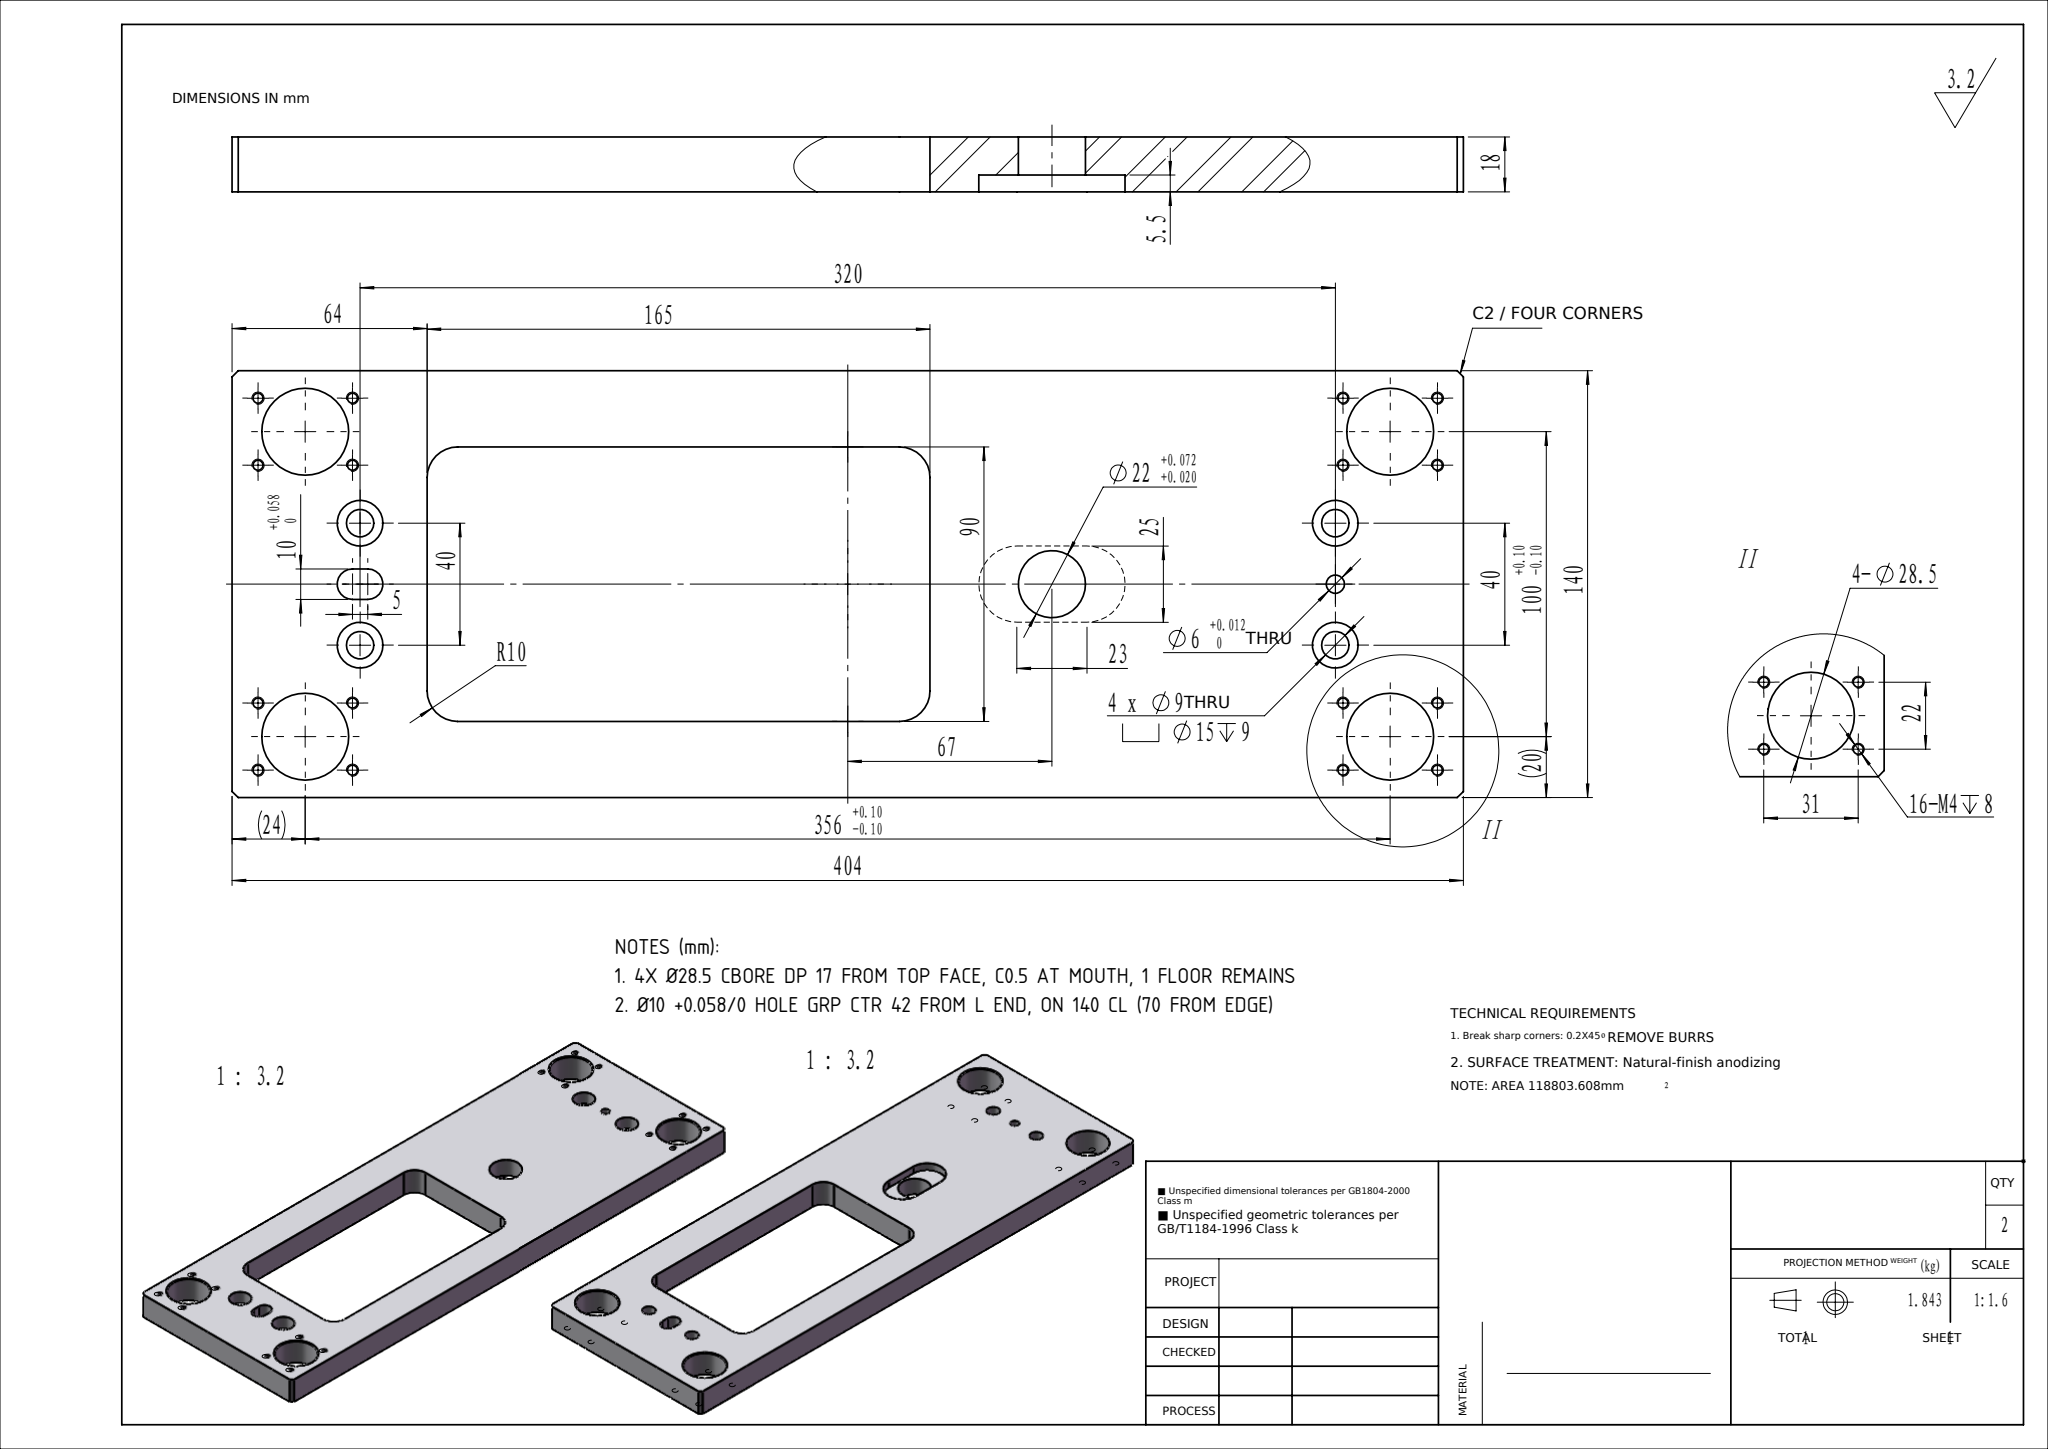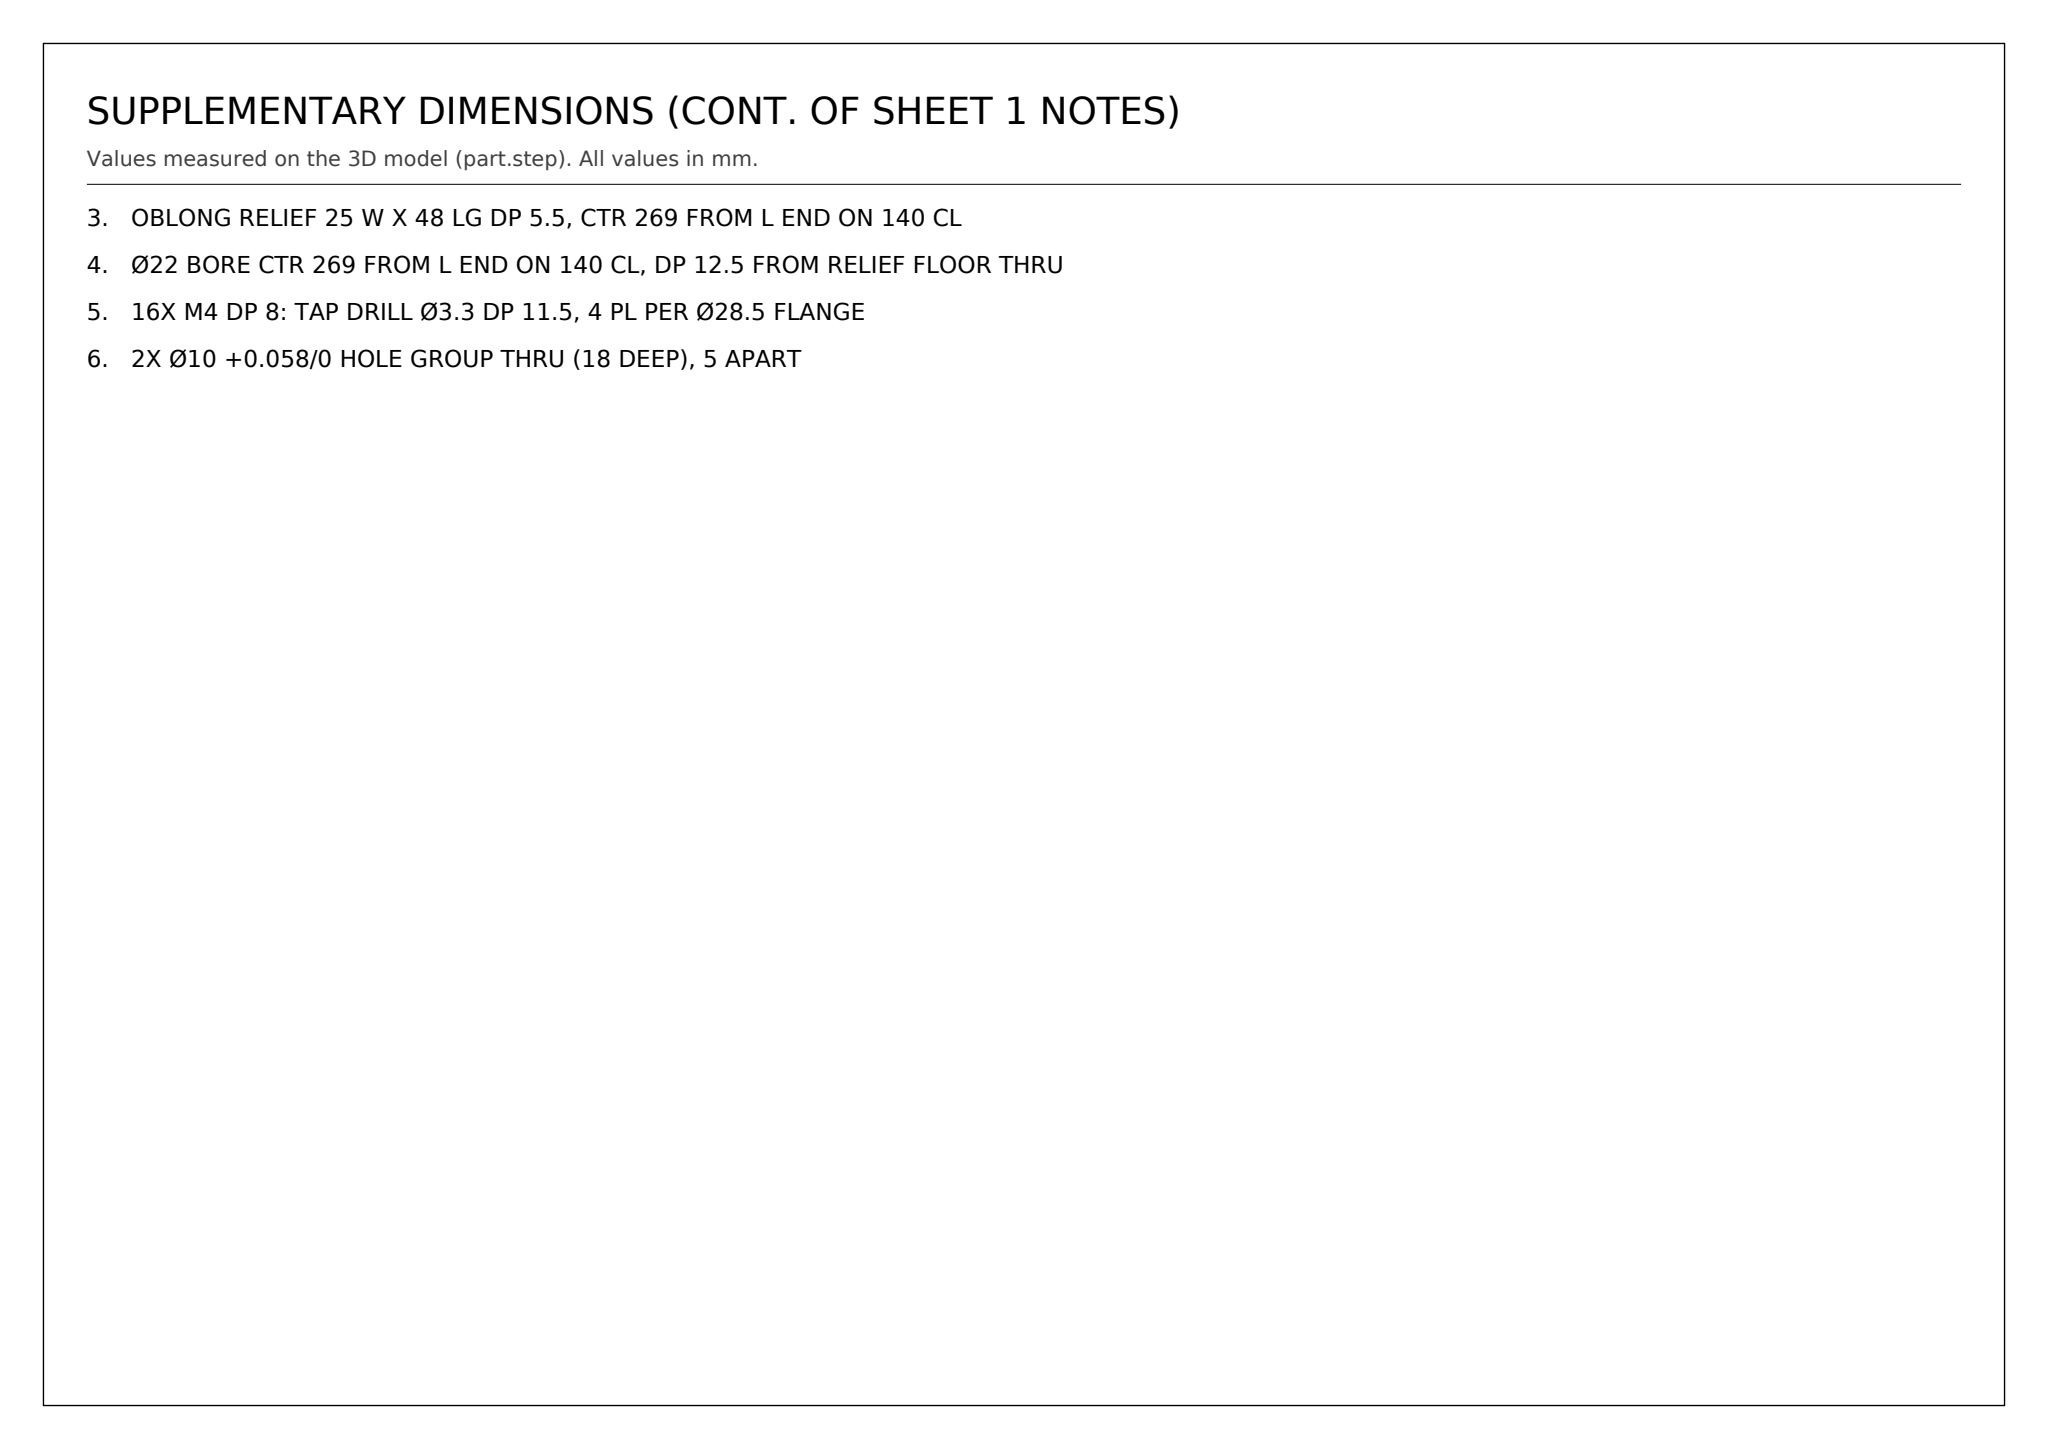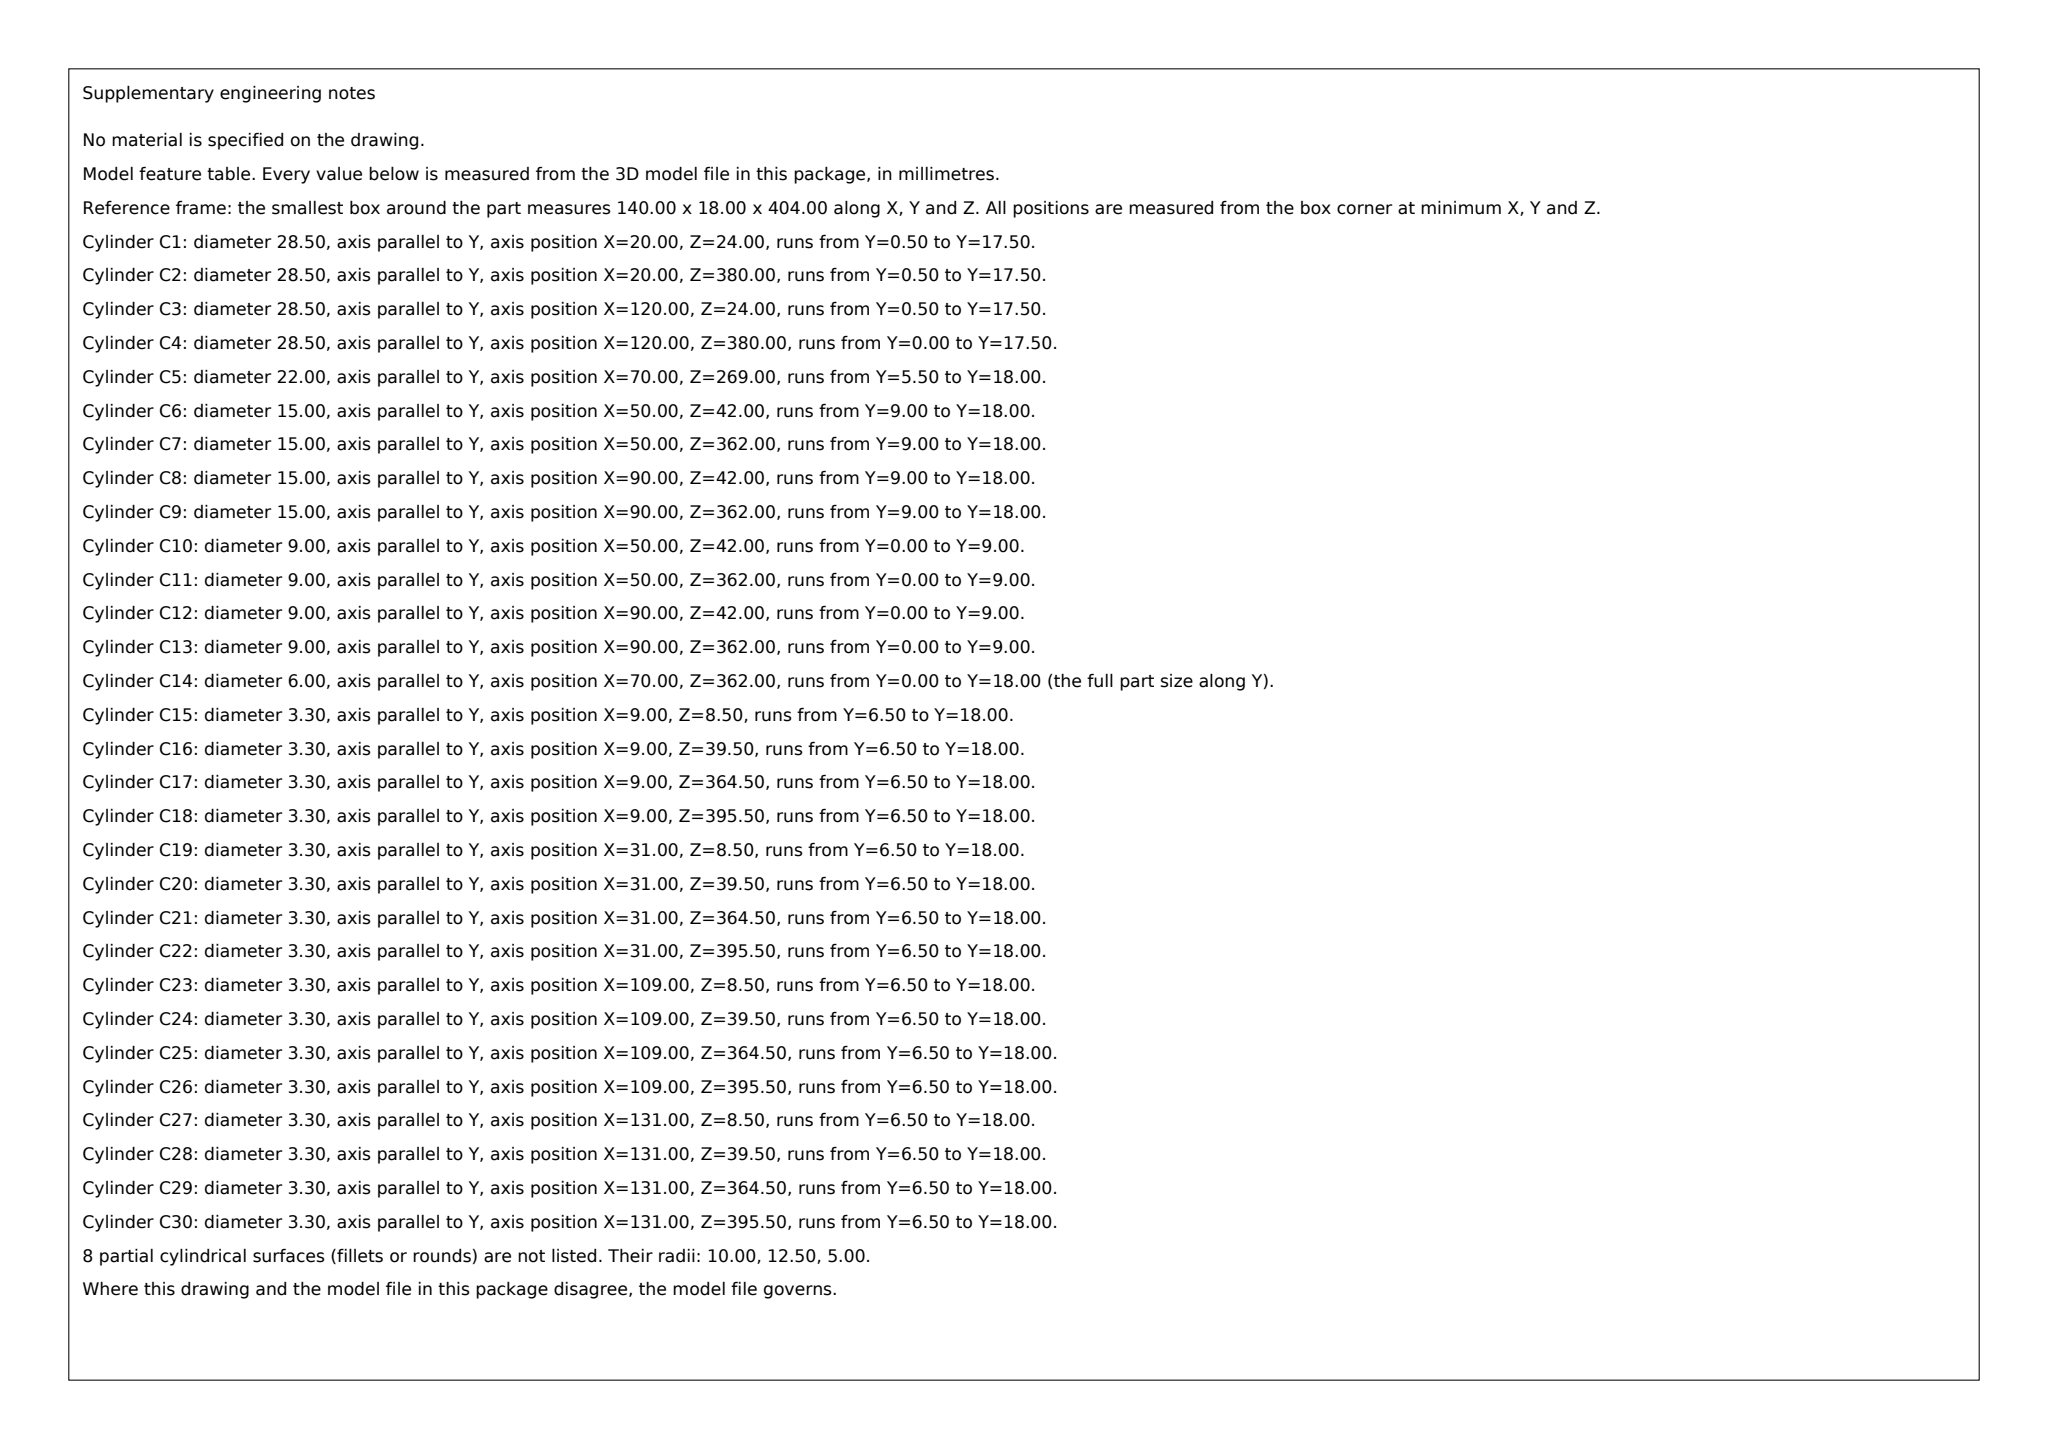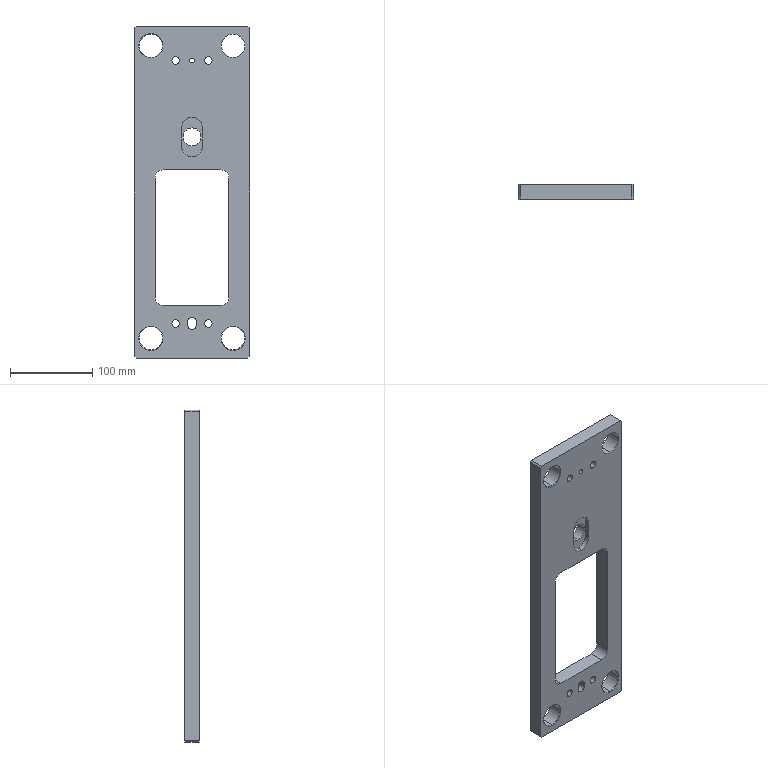Part | SolidWorks | mm | 1 solid | 139 faces | box 140 x 18 x 404 mm | volume 682463 mm3 | cylinder 70 | cone 46 | plane 23 | commonest cylinder face diameters 3.3 x32 15 x8 9 x8 28.5 x8 20 x4 25 x3 10 x3 6 x2
Drawing notes:
4X Ø28.5 CBORE DP 17 FROM TOP FACE, C0.5 AT MOUTH, 1 FLOOR REMAINS | from the solid: Ø28.5 cyls axis Y len 17.0 (one 17.5) at (20,24),(20,380),(120,24),(120,380) in 18 thk; 90° cone ref Ø29.5 = 0.5 csk
Ø10 +0.058/0 HOLE GRP CTR 42 FROM L END, ON 140 CL (70 FROM EDGE) | from the solid: Ø10 thru cyls (len 18) axis Y at x=70, z=39.5 & 44.5 -> grp ctr z=42, 5 apart; bbox 140 x 404
OBLONG RELIEF 25 W X 48 LG DP 5.5, CTR 269 FROM L END ON 140 CL | from the solid: Ø25 cyls len 5.5 at x=70, z=257.5 & 280.5 (23 apart, 23+25=48); plane y=5.5
Ø22 BORE CTR 269 FROM L END ON 140 CL, DP 12.5 FROM RELIEF FLOOR THRU | from the solid: Ø22 cyl len 12.5 at x=70, z=269; 5.5+12.5=18 = plate thk
16X M4 DP 8: TAP DRILL Ø3.3 DP 11.5, 4 PL PER Ø28.5 FLANGE | from the solid: Ø3.3 cyls len 11.5 at x=9/31 & 109/131, z=8.5/39.5 & 364.5/395.5; 118° drill point cones ref Ø3.3 x32
2X Ø10 +0.058/0 HOLE GROUP THRU (18 DEEP), 5 APART | from the solid: cylinders dia 10, axis y, pos [70,39.5] & [70,44.5], length 18 = full 18 plate thickness
build123d program:
from build123d import *

# Parameters (mm, degrees)
SKETCH1_W                                            = 140
SKETCH1_H                                            = 404
BOSS_EXTRUDE1_DEPTH                                  = 18
SKETCH2_R                                            = 14.25
CUT_EXTRUDE1_DEPTH                                   = 215.541
CHAMFER1_SIZE                                        = 2
M4_TAPPED_HOLE1_AT_2_COUNT                           = 2
M4_TAPPED_HOLE1_AT_2_PITCH                           = 22
M4_TAPPED_HOLE1_AT_3_COUNT                           = 2
M4_TAPPED_HOLE1_AT_3_PITCH                           = 31
M4_TAPPED_HOLE1_AT_4_COUNT                           = 2
M4_TAPPED_HOLE1_AT_4_PITCH                           = 38.013
HOLE_SIZE_ACCORDING_TO_THE_TYPE_OF_HEXAG_D           = 9
HOLE_SIZE_ACCORDING_TO_THE_TYPE_OF_HEXAG_CBORE_D     = 15
HOLE_SIZE_ACCORDING_TO_THE_TYPE_OF_HEXAG_CBORE_DEPTH = 9
F_6_0_6_DIAMETER_HOLE1_D                             = 6
CUT_EXTRUDE4_DEPTH                                   = 215.541
CHAMFER2_SIZE                                        = 0.5
SKETCH24_R                                           = 11
CUT_EXTRUDE8_DEPTH                                   = 215.541
CUT_EXTRUDE9_DEPTH                                   = 5.5
SKETCH26_W                                           = 90
SKETCH26_H                                           = 165
CUT_EXTRUDE10_DEPTH                                  = 215.541
FILLET2_R                                            = 10


with BuildPart() as part:
    # Sketch1 → Boss-Extrude1 (new body)
    with BuildSketch(Plane(origin=(0, 0, 0), x_dir=(1, 0, 0), z_dir=(0, 1, 0))):
        Rectangle(SKETCH1_W, SKETCH1_H)
    extrude(amount=BOSS_EXTRUDE1_DEPTH)

    # Sketch2 → Cut-Extrude1 (cut, through all)
    with BuildSketch(Plane(origin=(0, 18, 0), x_dir=(1, 0, 0), z_dir=(0, 1, 0))):
        with Locations(Location((-50, 178, 0), (0, 0, 270))):
            Circle(SKETCH2_R)
        with Locations(Location((50, 178, 0), (0, 0, 270))):
            Circle(SKETCH2_R)
        with Locations(Location((-50, -178, 0), (0, 0, 270))):
            Circle(SKETCH2_R)
        with Locations(Location((50, -178, 0), (0, 0, 270))):
            Circle(SKETCH2_R)
    extrude(amount=-CUT_EXTRUDE1_DEPTH, mode=Mode.SUBTRACT)

    # Chamfer1
    chamfer1_edges = [part.edges().sort_by_distance(p)[0] for p in [
        (70, 9, 202),
        (-70, 9, 202),
        (-70, 9, -202),
        (70, 9, -202),
    ]]
    chamfer(chamfer1_edges, length=CHAMFER1_SIZE)

    # Sketch7 → M4 Tapped Hole1 (revolve, cut)
    with BuildSketch(Plane(origin=(39, 18, 162.5), x_dir=(0, 0, 1), z_dir=(1, 0, 0))):
        Polygon((0, 0), (0, 12.491), (1.65, 11.5), (1.65, 0), align=None)
    m4_tapped_hole1 = revolve(axis=Axis((39, 24.35, 162.5), (0, -1, 0)), mode=Mode.SUBTRACT)

    # M4 Tapped Hole1 at 2: M4 Tapped Hole1 ×2
    with Locations(*[(i * M4_TAPPED_HOLE1_AT_2_PITCH, 0, 0) for i in range(1, M4_TAPPED_HOLE1_AT_2_COUNT)]):
        add(m4_tapped_hole1, mode=Mode.SUBTRACT)

    # M4 Tapped Hole1 at 3: M4 Tapped Hole1 ×2
    with Locations(*[(0, 0, i * M4_TAPPED_HOLE1_AT_3_PITCH) for i in range(1, M4_TAPPED_HOLE1_AT_3_COUNT)]):
        add(m4_tapped_hole1, mode=Mode.SUBTRACT)

    # M4 Tapped Hole1 at 4: M4 Tapped Hole1 ×2
    with Locations(*[Vector(0.5787, 0, 0.8155) * (i * M4_TAPPED_HOLE1_AT_4_PITCH) for i in range(1, M4_TAPPED_HOLE1_AT_4_COUNT)]):
        add(m4_tapped_hole1, mode=Mode.SUBTRACT)

    # Mirror1: M4 Tapped Hole1 across plane
    add(m4_tapped_hole1.mirror(Plane(origin=(0, 0, 0), x_dir=(1, 0, 0), z_dir=(0, 0, -1))), mode=Mode.SUBTRACT)

    # Mirror1 copy 1 sketch → Mirror1 copy 1 (revolve, cut)
    with BuildSketch(Plane(origin=(61, 18, -162.5), x_dir=(0, 0, -1), z_dir=(1, 0, 0))):
        Polygon((0, 0), (0, -12.491), (1.65, -11.5), (1.65, 0), align=None)
    revolve(axis=Axis((61, 24.35, -162.5), (0, 1, 0)), mode=Mode.SUBTRACT)

    # Mirror1 copy 2 sketch → Mirror1 copy 2 (revolve, cut)
    with BuildSketch(Plane(origin=(39, 18, -193.5), x_dir=(0, 0, -1), z_dir=(1, 0, 0))):
        Polygon((0, 0), (0, -12.491), (1.65, -11.5), (1.65, 0), align=None)
    revolve(axis=Axis((39, 24.35, -193.5), (0, 1, 0)), mode=Mode.SUBTRACT)

    # Mirror1 copy 3 sketch → Mirror1 copy 3 (revolve, cut)
    with BuildSketch(Plane(origin=(61, 18, -193.5), x_dir=(0, 0, -1), z_dir=(1, 0, 0))):
        Polygon((0, 0), (0, -12.491), (1.65, -11.5), (1.65, 0), align=None)
    revolve(axis=Axis((61, 24.35, -193.5), (0, 1, 0)), mode=Mode.SUBTRACT)

    # Mirror2: M4 Tapped Hole1 across plane
    add(m4_tapped_hole1.mirror(Plane(origin=(0, 0, 0), x_dir=(0, 0, 1), z_dir=(1, 0, 0))), mode=Mode.SUBTRACT)

    # Mirror2 copy 1 sketch → Mirror2 copy 1 (revolve, cut)
    with BuildSketch(Plane(origin=(-61, 18, 162.5), x_dir=(0, 0, 1), z_dir=(-1, 0, 0))):
        Polygon((0, 0), (0, -12.491), (1.65, -11.5), (1.65, 0), align=None)
    revolve(axis=Axis((-61, 24.35, 162.5), (0, 1, 0)), mode=Mode.SUBTRACT)

    # Mirror2 copy 2 sketch → Mirror2 copy 2 (revolve, cut)
    with BuildSketch(Plane(origin=(-39, 18, 193.5), x_dir=(0, 0, 1), z_dir=(-1, 0, 0))):
        Polygon((0, 0), (0, -12.491), (1.65, -11.5), (1.65, 0), align=None)
    revolve(axis=Axis((-39, 24.35, 193.5), (0, 1, 0)), mode=Mode.SUBTRACT)

    # Mirror2 copy 3 sketch → Mirror2 copy 3 (revolve, cut)
    with BuildSketch(Plane(origin=(-61, 18, 193.5), x_dir=(0, 0, 1), z_dir=(-1, 0, 0))):
        Polygon((0, 0), (0, -12.491), (1.65, -11.5), (1.65, 0), align=None)
    revolve(axis=Axis((-61, 24.35, 193.5), (0, 1, 0)), mode=Mode.SUBTRACT)

    # Mirror2 copy 4 sketch → Mirror2 copy 4 (revolve, cut)
    with BuildSketch(Plane(origin=(-39, 18, -162.5), x_dir=(0, 0, -1), z_dir=(-1, 0, 0))):
        Polygon((0, 0), (0, 12.491), (1.65, 11.5), (1.65, 0), align=None)
    revolve(axis=Axis((-39, 24.35, -162.5), (0, -1, 0)), mode=Mode.SUBTRACT)

    # Mirror2 copy 5 sketch → Mirror2 copy 5 (revolve, cut)
    with BuildSketch(Plane(origin=(-61, 18, -162.5), x_dir=(0, 0, -1), z_dir=(-1, 0, 0))):
        Polygon((0, 0), (0, 12.491), (1.65, 11.5), (1.65, 0), align=None)
    revolve(axis=Axis((-61, 24.35, -162.5), (0, -1, 0)), mode=Mode.SUBTRACT)

    # Mirror2 copy 6 sketch → Mirror2 copy 6 (revolve, cut)
    with BuildSketch(Plane(origin=(-39, 18, -193.5), x_dir=(0, 0, -1), z_dir=(-1, 0, 0))):
        Polygon((0, 0), (0, 12.491), (1.65, 11.5), (1.65, 0), align=None)
    revolve(axis=Axis((-39, 24.35, -193.5), (0, -1, 0)), mode=Mode.SUBTRACT)

    # Mirror2 copy 7 sketch → Mirror2 copy 7 (revolve, cut)
    with BuildSketch(Plane(origin=(-61, 18, -193.5), x_dir=(0, 0, -1), z_dir=(-1, 0, 0))):
        Polygon((0, 0), (0, 12.491), (1.65, 11.5), (1.65, 0), align=None)
    revolve(axis=Axis((-61, 24.35, -193.5), (0, -1, 0)), mode=Mode.SUBTRACT)

    # Hole Size according to the type of hexag (through all)
    with Locations(Plane(origin=(0, 18, 0), x_dir=(1, 0, 0), z_dir=(0, 1, 0))):
        with Locations((-20, 160), (20, 160), (-20, -160), (20, -160)):
            CounterBoreHole(HOLE_SIZE_ACCORDING_TO_THE_TYPE_OF_HEXAG_D / 2, HOLE_SIZE_ACCORDING_TO_THE_TYPE_OF_HEXAG_CBORE_D / 2, HOLE_SIZE_ACCORDING_TO_THE_TYPE_OF_HEXAG_CBORE_DEPTH)

    # 6.0 _6_ Diameter Hole1 (through all)
    with Locations(Plane(origin=(0, 18, 0), x_dir=(1, 0, 0), z_dir=(0, 1, 0))):
        with Locations((0, -160)):
            Hole(F_6_0_6_DIAMETER_HOLE1_D / 2)

    # Sketch19 → Cut-Extrude4 (cut, through all)
    with BuildSketch(Plane(origin=(0, 18, 0), x_dir=(1, 0, 0), z_dir=(0, 1, 0))):
        with BuildLine():
            Line((-5, 157.5), (-5, 162.5))
            ThreePointArc((-5, 162.5), (0, 167.5), (5, 162.5))
            Line((5, 162.5), (5, 157.5))
            ThreePointArc((5, 157.5), (0, 152.5), (-5, 157.5))
        make_face()
    extrude(amount=-CUT_EXTRUDE4_DEPTH, mode=Mode.SUBTRACT)

    # Chamfer2
    chamfer2_edges = [part.edges().sort_by_distance(p)[0] for p in [
        (-50, 0, -192.25),
        (-50, 18, -192.25),
        (50, 0, -192.25),
        (50, 18, -192.25),
        (-50, 0, 163.75),
        (-50, 18, 163.75),
        (50, 18, 163.75),
    ]]
    chamfer(chamfer2_edges, length=CHAMFER2_SIZE)

    # Sketch24 → Cut-Extrude8 (cut, through all)
    with BuildSketch(Plane(origin=(0, 18, 0), x_dir=(1, 0, 0), z_dir=(0, 1, 0))):
        with Locations(Location((0, -67, 0), (0, 0, 270))):
            Circle(SKETCH24_R)
    extrude(amount=-CUT_EXTRUDE8_DEPTH, mode=Mode.SUBTRACT)

    # Sketch25 → Cut-Extrude9 (cut)
    with BuildSketch(Plane.XZ):
        with BuildLine():
            Line((-12.5, 55.5), (-12.5, 78.5))
            ThreePointArc((-12.5, 78.5), (0, 91), (12.5, 78.5))
            Line((12.5, 78.5), (12.5, 55.5))
            ThreePointArc((12.5, 55.5), (0, 43), (-12.5, 55.5))
        make_face()
    extrude(amount=-CUT_EXTRUDE9_DEPTH, mode=Mode.SUBTRACT)

    # Sketch26 → Cut-Extrude10 (cut, through all)
    with BuildSketch(Plane.XZ):
        with Locations((0, -55.5)):
            Rectangle(SKETCH26_W, SKETCH26_H)
    extrude(amount=-CUT_EXTRUDE10_DEPTH, mode=Mode.SUBTRACT)

    # Fillet2
    fillet2_edges = [part.edges().sort_by_distance(p)[0] for p in [
        (45, 9, 27),
        (45, 9, -138),
        (-45, 9, -138),
        (-45, 9, 27),
    ]]
    fillet(fillet2_edges, radius=FILLET2_R)


solid = part.part